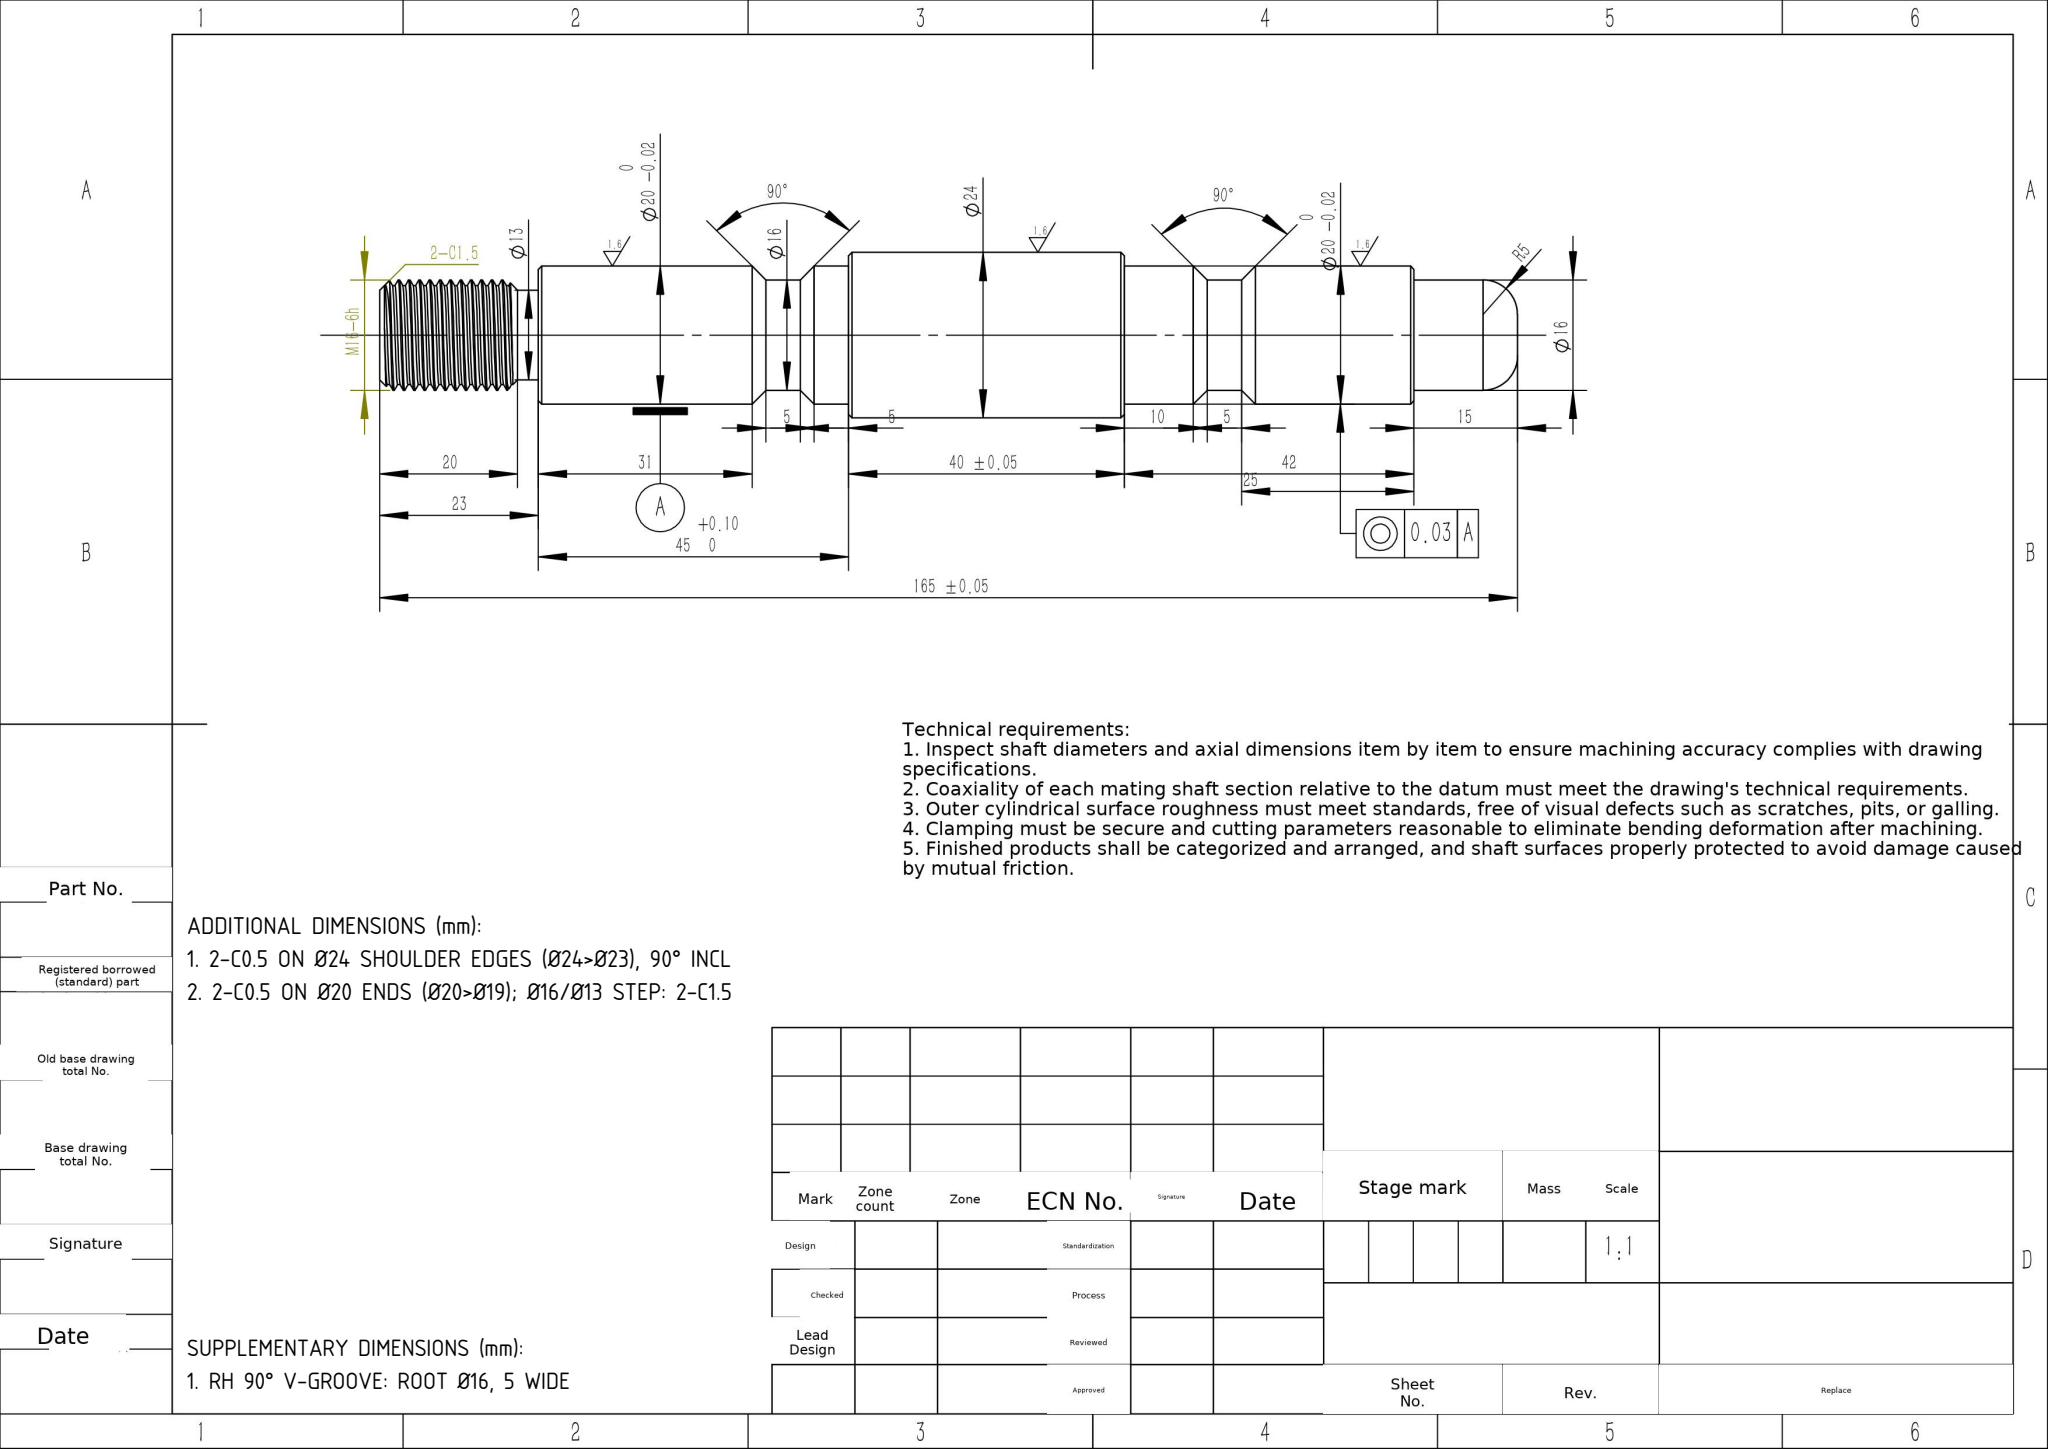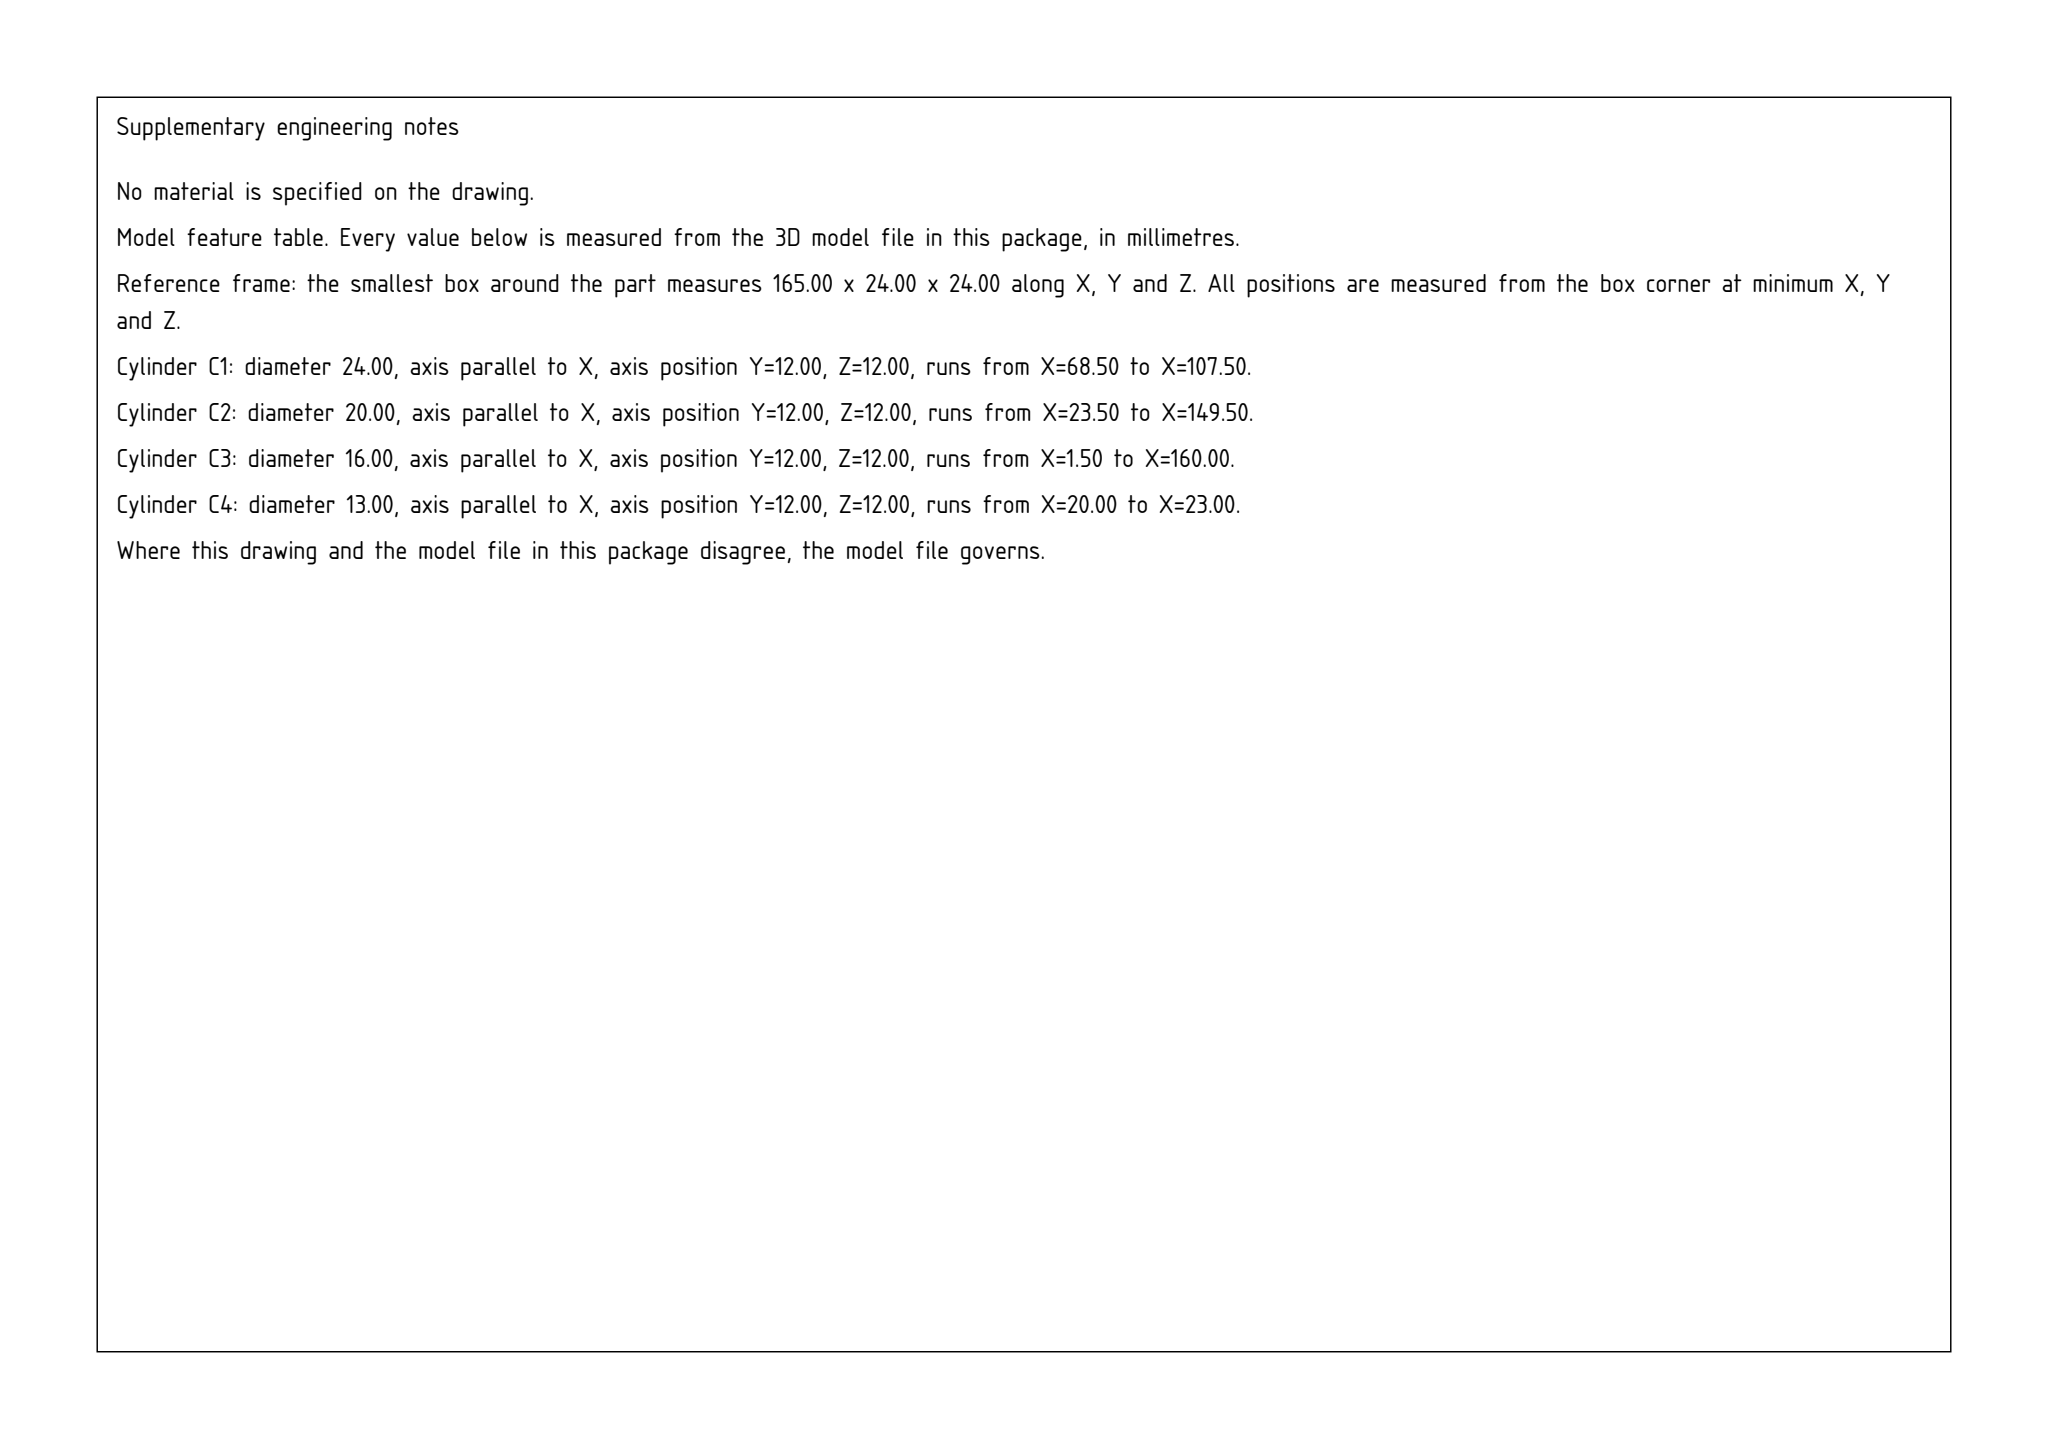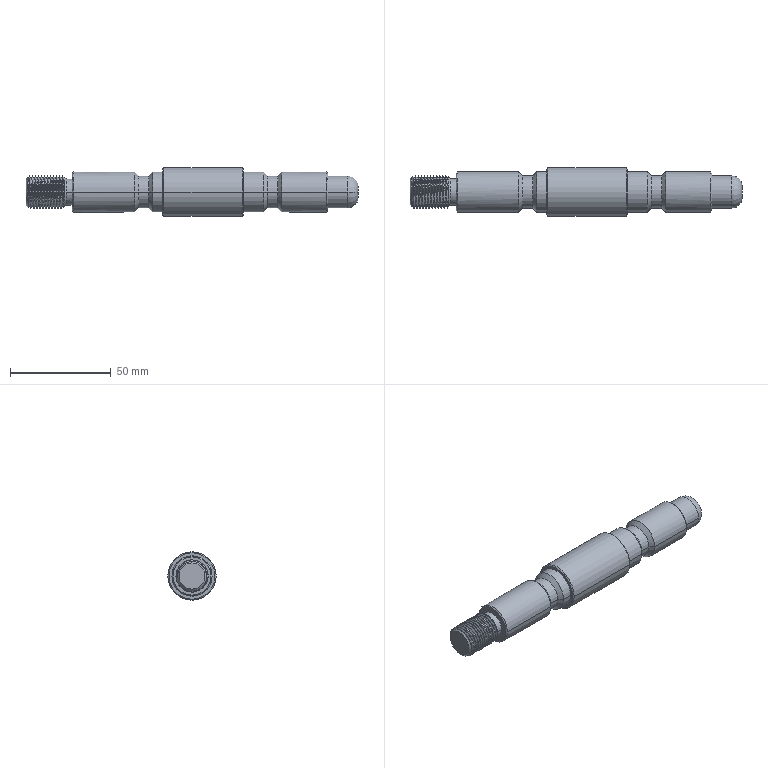Part | SolidWorks | mm | 1 solid | 73 faces | box 165 x 24 x 24 mm | volume 50476 mm3 | cylinder 42 | cone 20 | plane 6 | spline 3 | torus 2 | commonest cylinder face diameters 16 x30 20 x8 13 x2 24 x2